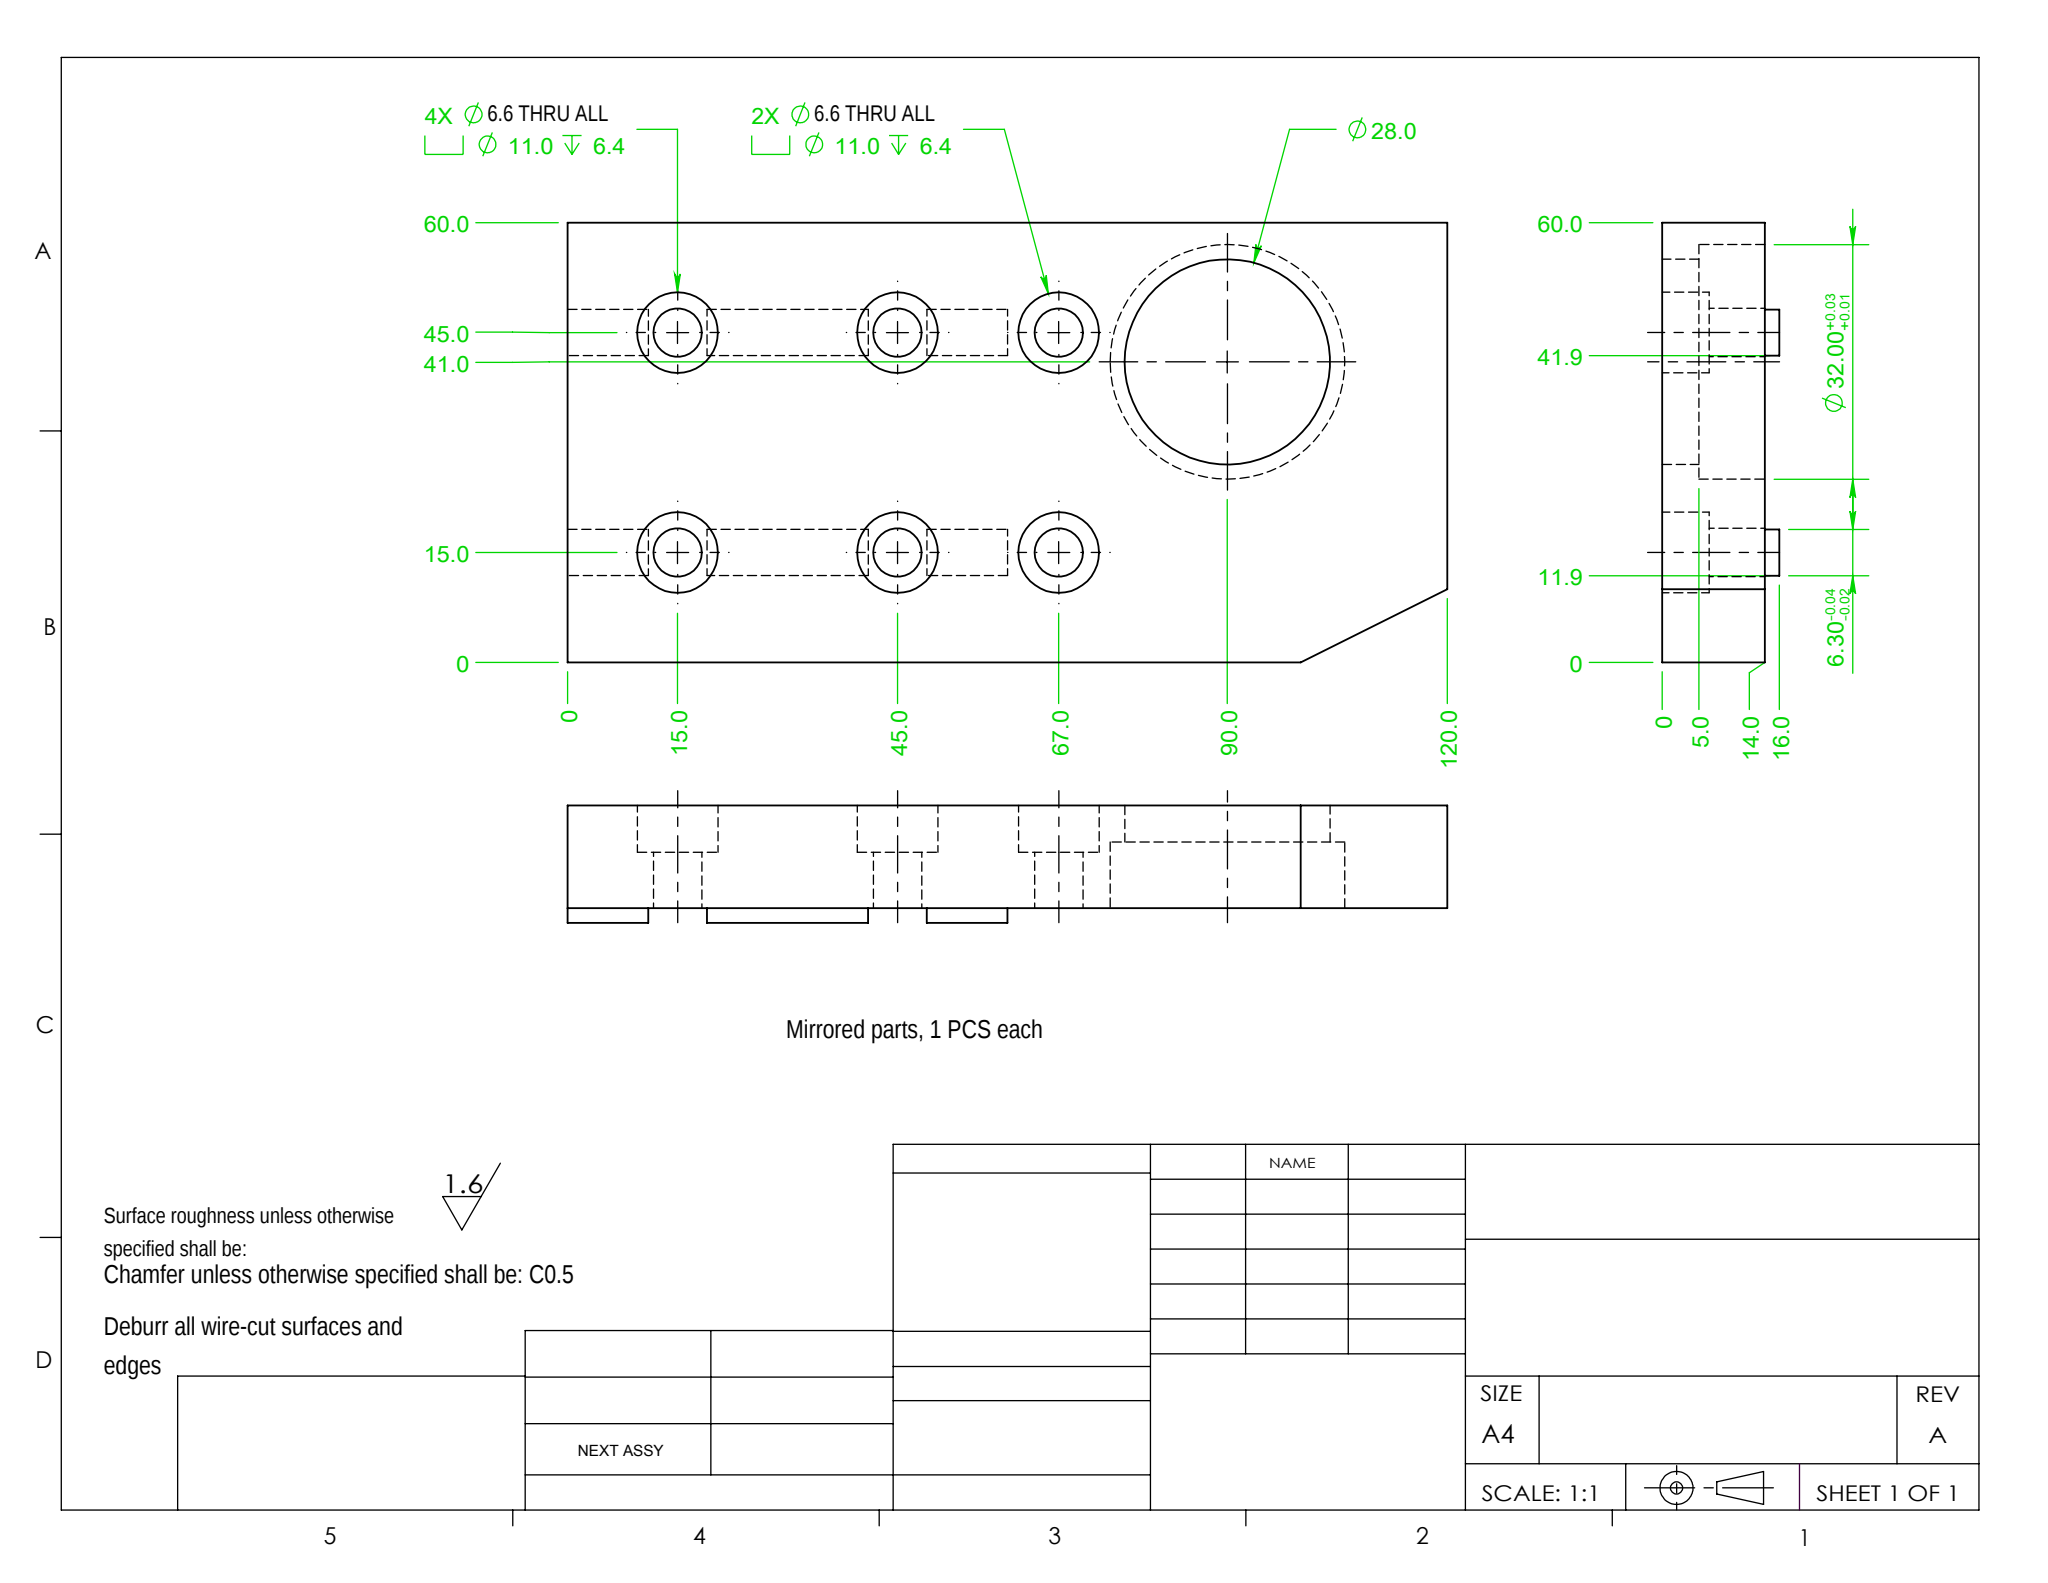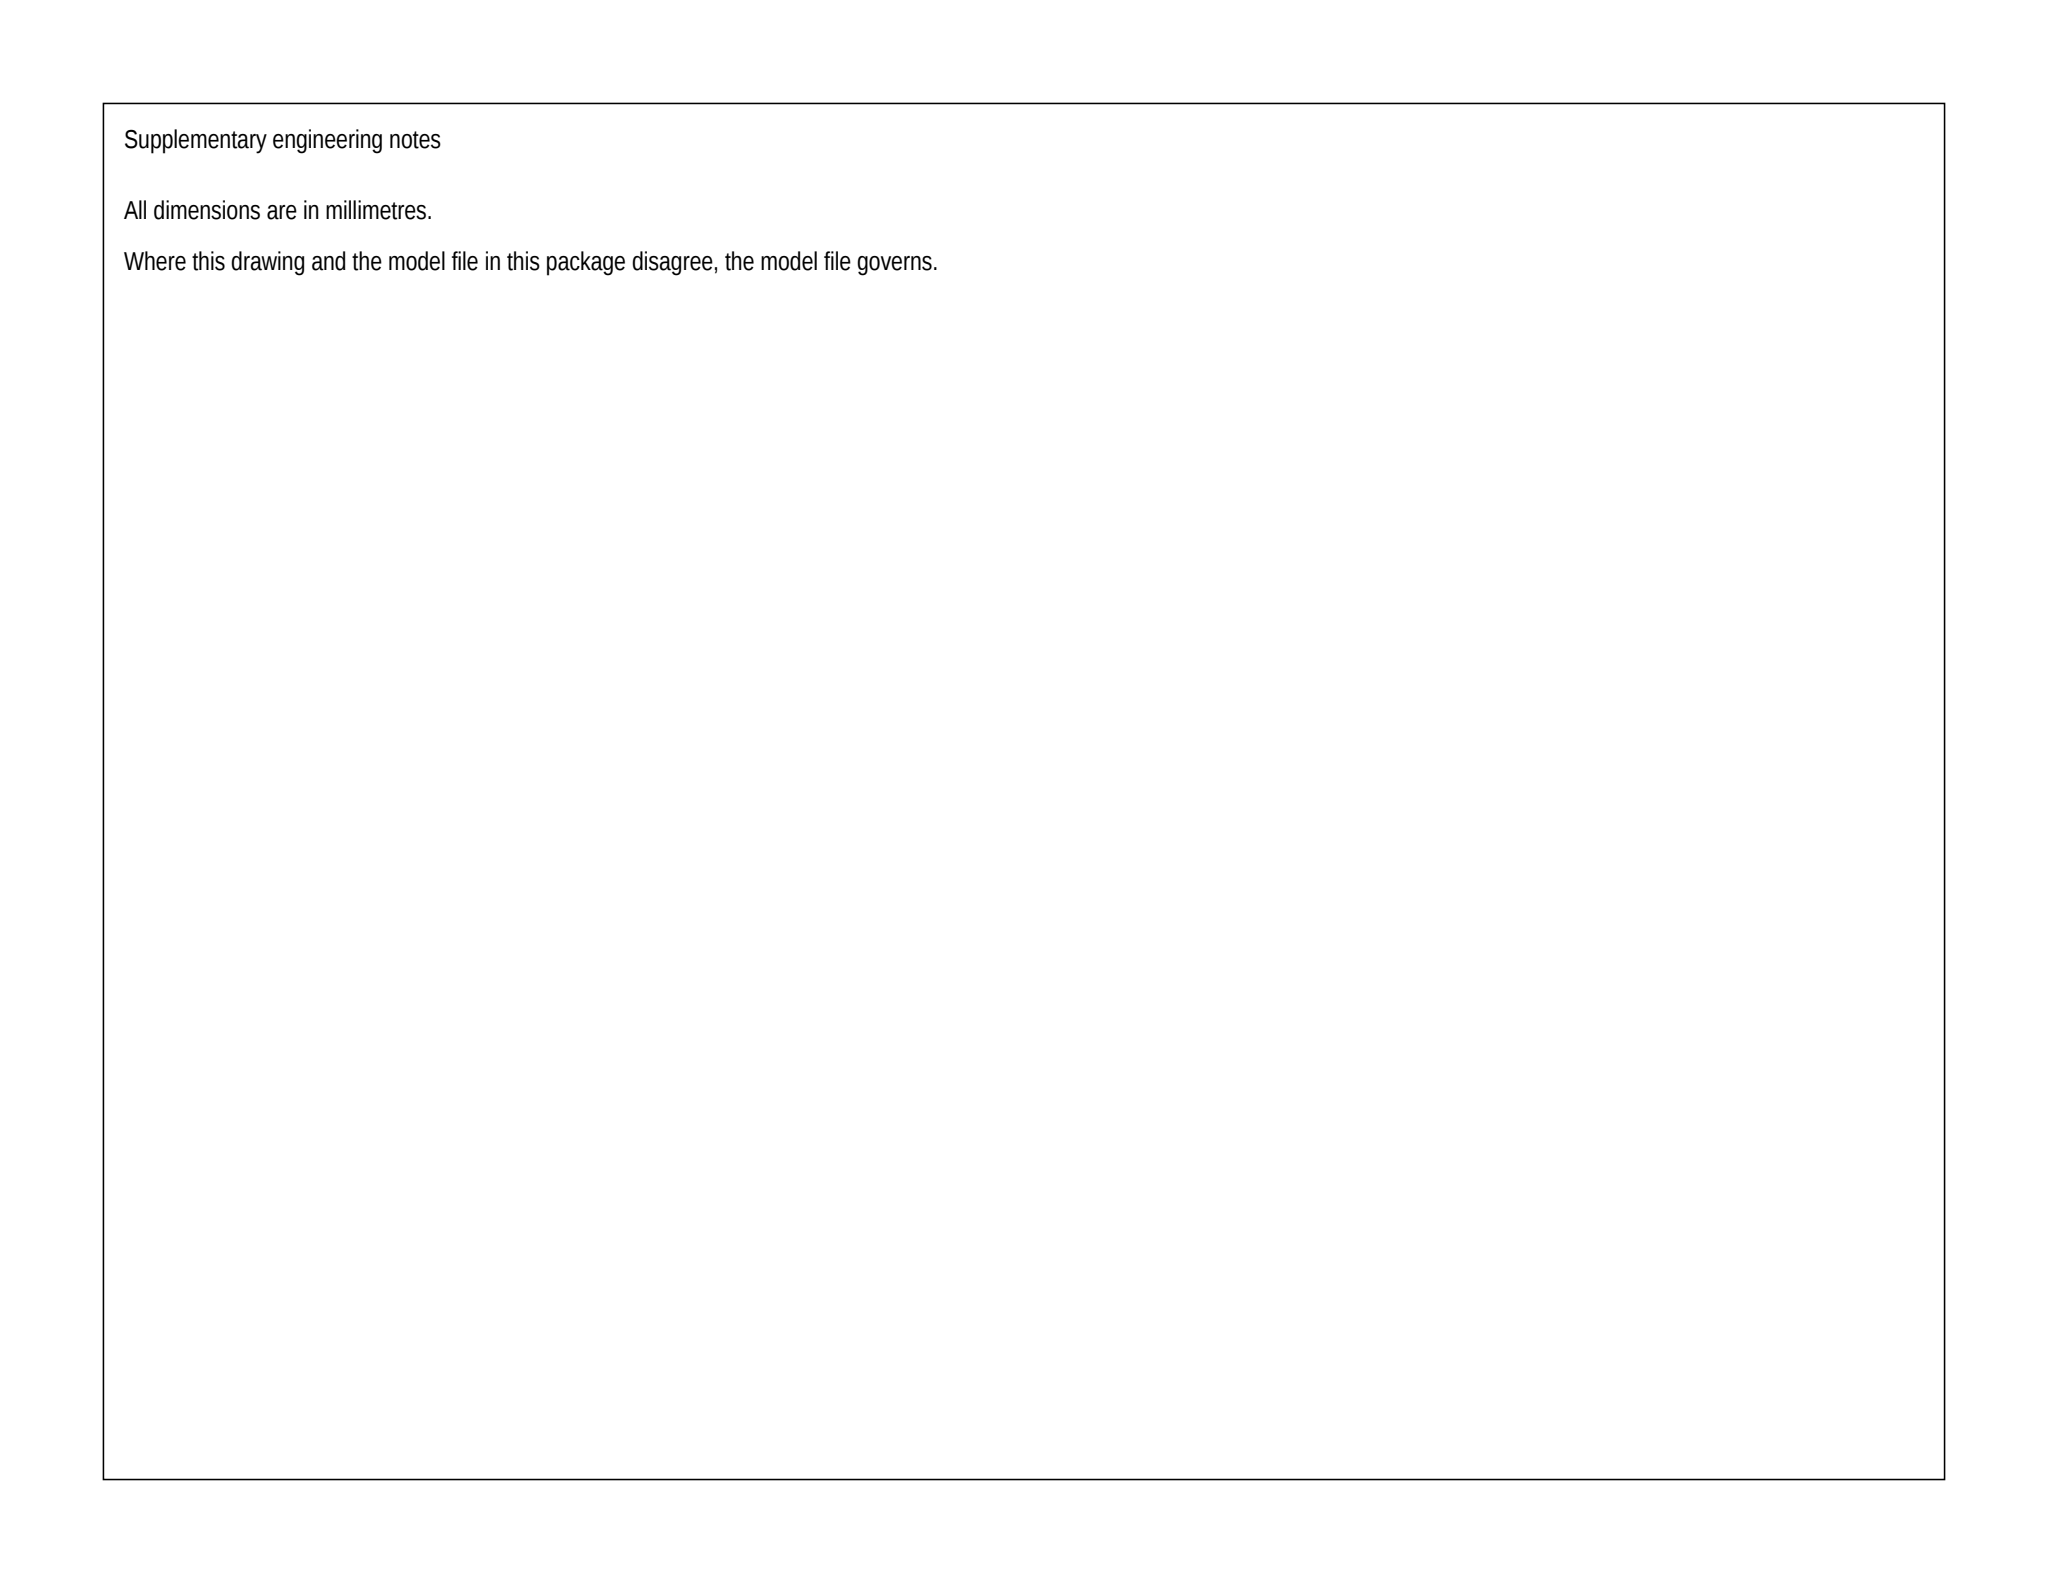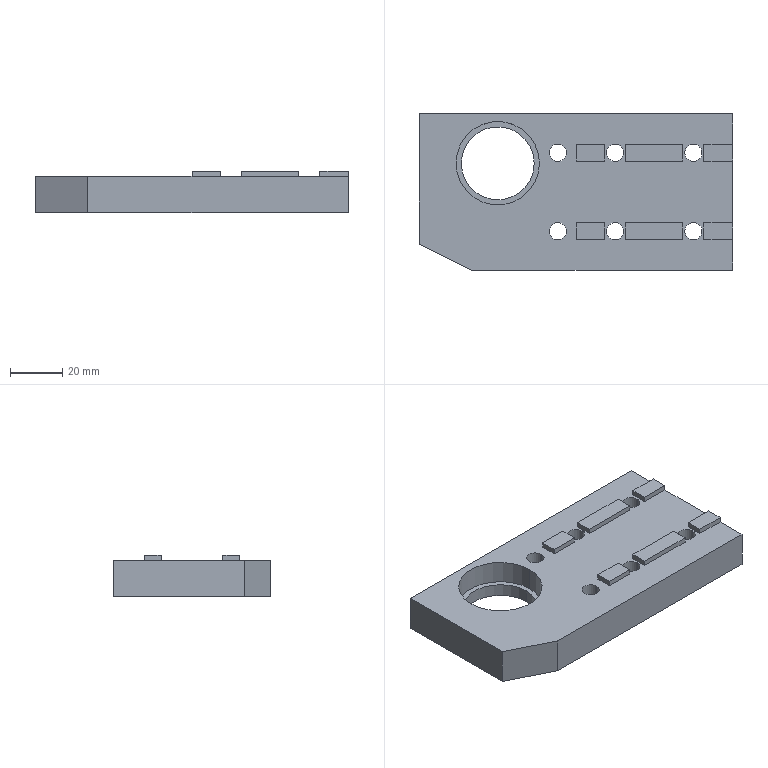Part | SolidWorks | mm | 1 solid | 70 faces | box 120 x 60 x 16 mm | volume 84982 mm3 | plane 42 | cylinder 28 | commonest cylinder face diameters 11 x12 6.6 x12 28 x2 32 x2
Drawing notes:
2X 6.3 WIDE RAIL (Y15 & Y45): 60.0 LG, ENDS 60.0 FROM LEFT EDGE | from the solid: y-planes 11.85/18.15 & 41.85/48.15 (6.3 wide); x-plane at 60.0 terminates rails spanning to part edge; bbox x=120.0
ITEM 1: CHAMFER 20.0 X 10.0 AT LOWER RH CORNER | from the solid: Bbox 120x60; corner cut between X planes 0/120 and Y plane 0 gives 20.0 x 10.0 corner chamfer
ITEM 2: SLOT FACE 11.0 FROM LH EDGE (X0) | from the solid: axis_plane x=109.0 -> 120.0-109.0 = 11.0 in mirrored drawing datum
ITEM 3: SLOT FACE 19.0 FROM LH EDGE (X0); SLOT 8.0 WIDE | from the solid: axis_plane x=101.0 -> 120.0-101.0 = 19.0; 19.0-11.0 = 8.0 wide
ITEM 4: SLOT FACE 41.0 FROM LH EDGE (X0) | from the solid: axis_plane x=79.0 -> 120.0-79.0 = 41.0
ITEM 5: SLOT FACE 49.0 FROM LH EDGE (X0); SLOT 8.0 WIDE | from the solid: axis_plane x=71.0 -> 120.0-71.0 = 49.0; 49.0-41.0 = 8.0 wide
build123d program:
from build123d import *

# Parameters (mm, degrees)
SKETCH1_W                                       = 120
SKETCH1_H                                       = 60
BOSS_EXTRUDE1_DEPTH                             = 14
CHAMFER1_SIZE                                   = 10
CHAMFER1_SIZE2                                  = 20
SKETCH4_W                                       = 60
SKETCH4_H                                       = 6.3
BOSS_EXTRUDE2_DEPTH                             = 2
M6_HEX_SOCKET_HEAD_CAP_SCREW_CBORE1_D           = 6.6
M6_HEX_SOCKET_HEAD_CAP_SCREW_CBORE1_CBORE_D     = 11
M6_HEX_SOCKET_HEAD_CAP_SCREW_CBORE1_CBORE_DEPTH = 6.4
SKETCH8_W                                       = 8
SKETCH8_H                                       = 60
CUT_EXTRUDE1_DEPTH                              = 2
SKETCH9_R                                       = 16
CUT_EXTRUDE2_DEPTH                              = 9
CUT_EXTRUDE3_DEPTH                              = 68.978
CUT_EXTRUDE3_DEPTH_BACK                         = 68.978
SKETCH10_R                                      = 14
M6_HEX_SOCKET_HEAD_CAP_SCREW_CBORE2_D           = 6.6
M6_HEX_SOCKET_HEAD_CAP_SCREW_CBORE2_CBORE_D     = 11
M6_HEX_SOCKET_HEAD_CAP_SCREW_CBORE2_CBORE_DEPTH = 6.4


with BuildPart() as part:
    # Sketch1 → Boss-Extrude1 (new body)
    with BuildSketch(Plane.XY):
        Rectangle(SKETCH1_W, SKETCH1_H)
    extrude(amount=BOSS_EXTRUDE1_DEPTH)

    # Chamfer1
    chamfer1_edges = [part.edges().sort_by_distance(p)[0] for p in [
        (-60, -30, 7),
    ]]
    chamfer1_side = [part.faces().sort_by_distance(p)[0] for p in [
        (-60, 0, 7),
    ]]
    chamfer(chamfer1_edges, length=CHAMFER1_SIZE, length2=CHAMFER1_SIZE2, reference=chamfer1_side[0])

    # Sketch4 → Boss-Extrude2 (add)
    with BuildSketch(Plane.XY.offset(14)):
        with Locations((30, -15)):
            Rectangle(SKETCH4_W, SKETCH4_H)
        with Locations((30, 15)):
            Rectangle(SKETCH4_W, SKETCH4_H)
    extrude(amount=BOSS_EXTRUDE2_DEPTH)

    # M6 Hex Socket Head Cap Screw CBORE1 (through all)
    with Locations(Plane(origin=(0, 0, 0), x_dir=(-1, 0, 0), z_dir=(0, 0, -1))):
        with Locations((-45, 15), (-15, 15), (-15, -15), (-45, -15)):
            CounterBoreHole(M6_HEX_SOCKET_HEAD_CAP_SCREW_CBORE1_D / 2, M6_HEX_SOCKET_HEAD_CAP_SCREW_CBORE1_CBORE_D / 2, M6_HEX_SOCKET_HEAD_CAP_SCREW_CBORE1_CBORE_DEPTH)

    # Sketch8 → Cut-Extrude1 (cut)
    with BuildSketch(Plane.XY.offset(16)):
        with Locations((15, 0)):
            Rectangle(SKETCH8_W, SKETCH8_H)
        with Locations((45, 0)):
            Rectangle(SKETCH8_W, SKETCH8_H)
    extrude(amount=-CUT_EXTRUDE1_DEPTH, mode=Mode.SUBTRACT)

    # Sketch9 → Cut-Extrude2 (cut)
    with BuildSketch(Plane.XY.offset(14)):
        with Locations((-30, 11)):
            Circle(SKETCH9_R)
    extrude(amount=-CUT_EXTRUDE2_DEPTH, mode=Mode.SUBTRACT)

    # Sketch10 → Cut-Extrude3 (cut, two sides: drawn at the far end of the back side and taken through both)
    with BuildSketch(Plane.XY.offset(5).offset(-CUT_EXTRUDE3_DEPTH_BACK)):
        with Locations((-30, 11)):
            Circle(SKETCH10_R)
    extrude(amount=CUT_EXTRUDE3_DEPTH + CUT_EXTRUDE3_DEPTH_BACK, mode=Mode.SUBTRACT)

    # M6 Hex Socket Head Cap Screw CBORE2 (through all)
    with Locations(Plane(origin=(0, 0, 0), x_dir=(-1, 0, 0), z_dir=(0, 0, -1))):
        with Locations((7, 15), (7, -15)):
            CounterBoreHole(M6_HEX_SOCKET_HEAD_CAP_SCREW_CBORE2_D / 2, M6_HEX_SOCKET_HEAD_CAP_SCREW_CBORE2_CBORE_D / 2, M6_HEX_SOCKET_HEAD_CAP_SCREW_CBORE2_CBORE_DEPTH)


solid = part.part